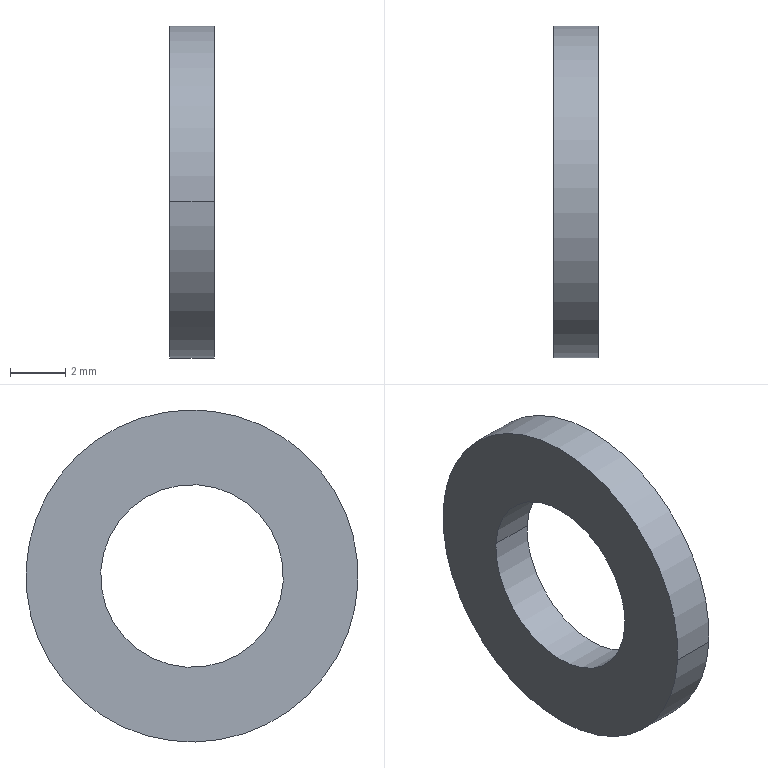Component | SolidWorks | plain washers--product grade c gb-5 | 1 solid | 6 faces | volume 126 mm3 | cylinder 4 | plane 2 | commonest cylinder face diameters 6.6 x2 12 x2